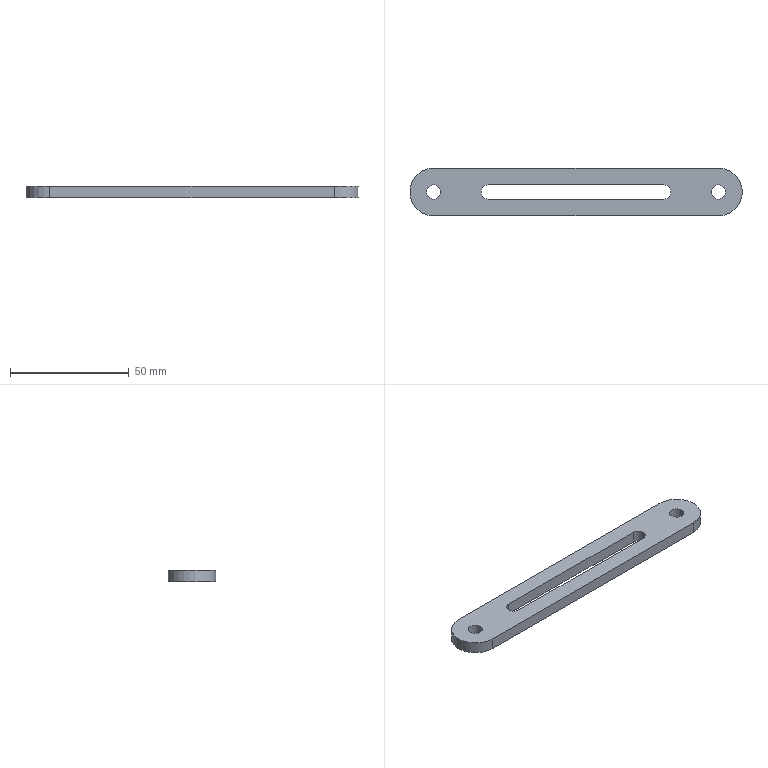Component | NX | LOWER_CONN_PLATE | 1 solid | 12 faces | box 140 x 20 x 5 mm | volume 10927 mm3 | plane 6 | cylinder 6 | commonest cylinder face diameters 6 x4 20 x2
STEP:
#1=CARTESIAN_POINT('',(0.,0.,0.));
#2=DIRECTION('',(0.,0.,1.));
#3=DIRECTION('',(1.,0.,0.));
#4=AXIS2_PLACEMENT_3D('',#1,#2,#3);
#5=CARTESIAN_POINT('',(-37.,3.,2.5));
#6=VERTEX_POINT('',#5);
#7=CARTESIAN_POINT('',(37.,3.,2.5));
#8=VERTEX_POINT('',#7);
#9=CARTESIAN_POINT('',(-40.,3.,2.5));
#10=DIRECTION('',(1.,0.,0.));
#11=VECTOR('',#10,1.);
#12=LINE('',#9,#11);
#13=CARTESIAN_POINT('',(-40.,3.,2.5));
#14=DIRECTION('',(0.,1.,0.));
#15=DIRECTION('',(0.,0.,1.));
#16=AXIS2_PLACEMENT_3D('',#13,#14,#15);
#17=PLANE('',#16);
#18=CARTESIAN_POINT('',(0.,0.));
#19=DIRECTION('',(0.,1.));
#20=VECTOR('',#19,1.);
#21=LINE('',#18,#20);
#22=(GEOMETRIC_REPRESENTATION_CONTEXT(2)PARAMETRIC_REPRESENTATION_CONTEXT()REPRESENTATION_CONTEXT('',''));
#23=DEFINITIONAL_REPRESENTATION('',(#21),#22);
#24=PCURVE('',#17,#23);
#25=CARTESIAN_POINT('',(-60.,0.,2.5));
#26=DIRECTION('',(0.,0.,1.));
#27=DIRECTION('',(1.,0.,0.));
#28=AXIS2_PLACEMENT_3D('',#25,#26,#27);
#29=PLANE('',#28);
#30=CARTESIAN_POINT('',(20.,3.));
#31=DIRECTION('',(1.,0.));
#32=VECTOR('',#31,1.);
#33=LINE('',#30,#32);
#34=(GEOMETRIC_REPRESENTATION_CONTEXT(2)PARAMETRIC_REPRESENTATION_CONTEXT()REPRESENTATION_CONTEXT('',''));
#35=DEFINITIONAL_REPRESENTATION('',(#33),#34);
#36=PCURVE('',#29,#35);
#37=SURFACE_CURVE('',#12,(#24,#36),.PCURVE_S1.);
#38=EDGE_CURVE('',#6,#8,#37,.T.);
#39=ORIENTED_EDGE('',*,*,#38,.F.);
#40=CARTESIAN_POINT('',(-37.,3.,-2.5));
#41=VERTEX_POINT('',#40);
#42=CARTESIAN_POINT('',(-37.,3.,-2.5));
#43=DIRECTION('',(0.,0.,-1.));
#44=VECTOR('',#43,1.);
#45=LINE('',#42,#44);
#46=CARTESIAN_POINT('',(-5.,3.));
#47=DIRECTION('',(-1.,0.));
#48=VECTOR('',#47,1.);
#49=LINE('',#46,#48);
#50=(GEOMETRIC_REPRESENTATION_CONTEXT(2)PARAMETRIC_REPRESENTATION_CONTEXT()REPRESENTATION_CONTEXT('',''));
#51=DEFINITIONAL_REPRESENTATION('',(#49),#50);
#52=PCURVE('',#17,#51);
#53=CARTESIAN_POINT('',(-37.,0.,2.5));
#54=DIRECTION('',(0.,0.,1.));
#55=DIRECTION('',(1.,0.,0.));
#56=AXIS2_PLACEMENT_3D('',#53,#54,#55);
#57=CYLINDRICAL_SURFACE('',#56,3.);
#58=CARTESIAN_POINT('',(1.571,-5.));
#59=DIRECTION('',(0.,-1.));
#60=VECTOR('',#59,1.);
#61=LINE('',#58,#60);
#62=(GEOMETRIC_REPRESENTATION_CONTEXT(2)PARAMETRIC_REPRESENTATION_CONTEXT()REPRESENTATION_CONTEXT('',''));
#63=DEFINITIONAL_REPRESENTATION('',(#61),#62);
#64=PCURVE('',#57,#63);
#65=SURFACE_CURVE('',#45,(#52,#64),.PCURVE_S1.);
#66=EDGE_CURVE('',#6,#41,#65,.T.);
#67=ORIENTED_EDGE('',*,*,#66,.T.);
#68=CARTESIAN_POINT('',(37.,3.,-2.5));
#69=VERTEX_POINT('',#68);
#70=CARTESIAN_POINT('',(-40.,3.,-2.5));
#71=DIRECTION('',(1.,0.,0.));
#72=VECTOR('',#71,1.);
#73=LINE('',#70,#72);
#74=CARTESIAN_POINT('',(-5.,0.));
#75=DIRECTION('',(0.,1.));
#76=VECTOR('',#75,1.);
#77=LINE('',#74,#76);
#78=(GEOMETRIC_REPRESENTATION_CONTEXT(2)PARAMETRIC_REPRESENTATION_CONTEXT()REPRESENTATION_CONTEXT('',''));
#79=DEFINITIONAL_REPRESENTATION('',(#77),#78);
#80=PCURVE('',#17,#79);
#81=CARTESIAN_POINT('',(-60.,0.,-2.5));
#82=DIRECTION('',(0.,0.,1.));
#83=DIRECTION('',(1.,0.,0.));
#84=AXIS2_PLACEMENT_3D('',#81,#82,#83);
#85=PLANE('',#84);
#86=CARTESIAN_POINT('',(20.,3.));
#87=DIRECTION('',(1.,0.));
#88=VECTOR('',#87,1.);
#89=LINE('',#86,#88);
#90=(GEOMETRIC_REPRESENTATION_CONTEXT(2)PARAMETRIC_REPRESENTATION_CONTEXT()REPRESENTATION_CONTEXT('',''));
#91=DEFINITIONAL_REPRESENTATION('',(#89),#90);
#92=PCURVE('',#85,#91);
#93=SURFACE_CURVE('',#73,(#80,#92),.PCURVE_S1.);
#94=EDGE_CURVE('',#41,#69,#93,.T.);
#95=ORIENTED_EDGE('',*,*,#94,.T.);
#96=CARTESIAN_POINT('',(37.,3.,2.5));
#97=DIRECTION('',(0.,0.,1.));
#98=VECTOR('',#97,1.);
#99=LINE('',#96,#98);
#100=CARTESIAN_POINT('',(0.,77.));
#101=DIRECTION('',(1.,0.));
#102=VECTOR('',#101,1.);
#103=LINE('',#100,#102);
#104=(GEOMETRIC_REPRESENTATION_CONTEXT(2)PARAMETRIC_REPRESENTATION_CONTEXT()REPRESENTATION_CONTEXT('',''));
#105=DEFINITIONAL_REPRESENTATION('',(#103),#104);
#106=PCURVE('',#17,#105);
#107=CARTESIAN_POINT('',(37.,0.,2.5));
#108=DIRECTION('',(0.,0.,1.));
#109=DIRECTION('',(1.,0.,0.));
#110=AXIS2_PLACEMENT_3D('',#107,#108,#109);
#111=CYLINDRICAL_SURFACE('',#110,3.);
#112=CARTESIAN_POINT('',(1.571,0.));
#113=DIRECTION('',(0.,1.));
#114=VECTOR('',#113,1.);
#115=LINE('',#112,#114);
#116=(GEOMETRIC_REPRESENTATION_CONTEXT(2)PARAMETRIC_REPRESENTATION_CONTEXT()REPRESENTATION_CONTEXT('',''));
#117=DEFINITIONAL_REPRESENTATION('',(#115),#116);
#118=PCURVE('',#111,#117);
#119=SURFACE_CURVE('',#99,(#106,#118),.PCURVE_S1.);
#120=EDGE_CURVE('',#69,#8,#119,.T.);
#121=ORIENTED_EDGE('',*,*,#120,.T.);
#122=EDGE_LOOP('',(#39,#67,#95,#121));
#123=FACE_BOUND('',#122,.T.);
#124=ADVANCED_FACE('',(#123),#17,.F.);
#125=CARTESIAN_POINT('',(-60.,-10.,-2.5));
#126=VERTEX_POINT('',#125);
#127=CARTESIAN_POINT('',(60.,-10.,-2.5));
#128=VERTEX_POINT('',#127);
#129=CARTESIAN_POINT('',(-70.,-10.,-2.5));
#130=DIRECTION('',(1.,0.,0.));
#131=VECTOR('',#130,1.);
#132=LINE('',#129,#131);
#133=CARTESIAN_POINT('',(-70.,-10.,2.5));
#134=DIRECTION('',(0.,1.,0.));
#135=DIRECTION('',(0.,0.,1.));
#136=AXIS2_PLACEMENT_3D('',#133,#134,#135);
#137=PLANE('',#136);
#138=CARTESIAN_POINT('',(-5.,0.));
#139=DIRECTION('',(0.,1.));
#140=VECTOR('',#139,1.);
#141=LINE('',#138,#140);
#142=(GEOMETRIC_REPRESENTATION_CONTEXT(2)PARAMETRIC_REPRESENTATION_CONTEXT()REPRESENTATION_CONTEXT('',''));
#143=DEFINITIONAL_REPRESENTATION('',(#141),#142);
#144=PCURVE('',#137,#143);
#145=CARTESIAN_POINT('',(-10.,-10.));
#146=DIRECTION('',(1.,0.));
#147=VECTOR('',#146,1.);
#148=LINE('',#145,#147);
#149=(GEOMETRIC_REPRESENTATION_CONTEXT(2)PARAMETRIC_REPRESENTATION_CONTEXT()REPRESENTATION_CONTEXT('',''));
#150=DEFINITIONAL_REPRESENTATION('',(#148),#149);
#151=PCURVE('',#85,#150);
#152=SURFACE_CURVE('',#132,(#144,#151),.PCURVE_S1.);
#153=EDGE_CURVE('',#126,#128,#152,.T.);
#154=ORIENTED_EDGE('',*,*,#153,.T.);
#155=CARTESIAN_POINT('',(60.,-10.,2.5));
#156=VERTEX_POINT('',#155);
#157=CARTESIAN_POINT('',(60.,-10.,2.5));
#158=DIRECTION('',(0.,0.,1.));
#159=VECTOR('',#158,1.);
#160=LINE('',#157,#159);
#161=CARTESIAN_POINT('',(0.,130.));
#162=DIRECTION('',(1.,0.));
#163=VECTOR('',#162,1.);
#164=LINE('',#161,#163);
#165=(GEOMETRIC_REPRESENTATION_CONTEXT(2)PARAMETRIC_REPRESENTATION_CONTEXT()REPRESENTATION_CONTEXT('',''));
#166=DEFINITIONAL_REPRESENTATION('',(#164),#165);
#167=PCURVE('',#137,#166);
#168=CARTESIAN_POINT('',(60.,0.,2.5));
#169=DIRECTION('',(0.,0.,-1.));
#170=DIRECTION('',(-1.,0.,0.));
#171=AXIS2_PLACEMENT_3D('',#168,#169,#170);
#172=CYLINDRICAL_SURFACE('',#171,10.);
#173=CARTESIAN_POINT('',(4.712,0.));
#174=DIRECTION('',(0.,-1.));
#175=VECTOR('',#174,1.);
#176=LINE('',#173,#175);
#177=(GEOMETRIC_REPRESENTATION_CONTEXT(2)PARAMETRIC_REPRESENTATION_CONTEXT()REPRESENTATION_CONTEXT('',''));
#178=DEFINITIONAL_REPRESENTATION('',(#176),#177);
#179=PCURVE('',#172,#178);
#180=SURFACE_CURVE('',#160,(#167,#179),.PCURVE_S1.);
#181=EDGE_CURVE('',#128,#156,#180,.T.);
#182=ORIENTED_EDGE('',*,*,#181,.T.);
#183=CARTESIAN_POINT('',(-60.,-10.,2.5));
#184=VERTEX_POINT('',#183);
#185=CARTESIAN_POINT('',(-70.,-10.,2.5));
#186=DIRECTION('',(1.,0.,0.));
#187=VECTOR('',#186,1.);
#188=LINE('',#185,#187);
#189=CARTESIAN_POINT('',(0.,0.));
#190=DIRECTION('',(0.,1.));
#191=VECTOR('',#190,1.);
#192=LINE('',#189,#191);
#193=(GEOMETRIC_REPRESENTATION_CONTEXT(2)PARAMETRIC_REPRESENTATION_CONTEXT()REPRESENTATION_CONTEXT('',''));
#194=DEFINITIONAL_REPRESENTATION('',(#192),#193);
#195=PCURVE('',#137,#194);
#196=CARTESIAN_POINT('',(-10.,-10.));
#197=DIRECTION('',(1.,0.));
#198=VECTOR('',#197,1.);
#199=LINE('',#196,#198);
#200=(GEOMETRIC_REPRESENTATION_CONTEXT(2)PARAMETRIC_REPRESENTATION_CONTEXT()REPRESENTATION_CONTEXT('',''));
#201=DEFINITIONAL_REPRESENTATION('',(#199),#200);
#202=PCURVE('',#29,#201);
#203=SURFACE_CURVE('',#188,(#195,#202),.PCURVE_S1.);
#204=EDGE_CURVE('',#184,#156,#203,.T.);
#205=ORIENTED_EDGE('',*,*,#204,.F.);
#206=CARTESIAN_POINT('',(-60.,-10.,2.5));
#207=DIRECTION('',(0.,0.,-1.));
#208=VECTOR('',#207,1.);
#209=LINE('',#206,#208);
#210=CARTESIAN_POINT('',(0.,10.));
#211=DIRECTION('',(-1.,0.));
#212=VECTOR('',#211,1.);
#213=LINE('',#210,#212);
#214=(GEOMETRIC_REPRESENTATION_CONTEXT(2)PARAMETRIC_REPRESENTATION_CONTEXT()REPRESENTATION_CONTEXT('',''));
#215=DEFINITIONAL_REPRESENTATION('',(#213),#214);
#216=PCURVE('',#137,#215);
#217=CARTESIAN_POINT('',(-60.,0.,2.5));
#218=DIRECTION('',(0.,0.,-1.));
#219=DIRECTION('',(-1.,0.,0.));
#220=AXIS2_PLACEMENT_3D('',#217,#218,#219);
#221=CYLINDRICAL_SURFACE('',#220,10.);
#222=CARTESIAN_POINT('',(4.712,0.));
#223=DIRECTION('',(0.,1.));
#224=VECTOR('',#223,1.);
#225=LINE('',#222,#224);
#226=(GEOMETRIC_REPRESENTATION_CONTEXT(2)PARAMETRIC_REPRESENTATION_CONTEXT()REPRESENTATION_CONTEXT('',''));
#227=DEFINITIONAL_REPRESENTATION('',(#225),#226);
#228=PCURVE('',#221,#227);
#229=SURFACE_CURVE('',#209,(#216,#228),.PCURVE_S1.);
#230=EDGE_CURVE('',#184,#126,#229,.T.);
#231=ORIENTED_EDGE('',*,*,#230,.T.);
#232=EDGE_LOOP('',(#154,#182,#205,#231));
#233=FACE_BOUND('',#232,.T.);
#234=ADVANCED_FACE('',(#233),#137,.F.);
#235=CARTESIAN_POINT('',(63.,0.,2.5));
#236=VERTEX_POINT('',#235);
#237=CARTESIAN_POINT('',(60.,0.,2.5));
#238=DIRECTION('',(0.,0.,1.));
#239=DIRECTION('',(1.,0.,0.));
#240=AXIS2_PLACEMENT_3D('',#237,#238,#239);
#241=CIRCLE('',#240,3.);
#242=CARTESIAN_POINT('',(60.,0.,2.5));
#243=DIRECTION('',(0.,0.,-1.));
#244=DIRECTION('',(-1.,0.,0.));
#245=AXIS2_PLACEMENT_3D('',#242,#243,#244);
#246=CYLINDRICAL_SURFACE('',#245,3.);
#247=CARTESIAN_POINT('',(9.425,0.));
#248=DIRECTION('',(-1.,0.));
#249=VECTOR('',#248,1.);
#250=LINE('',#247,#249);
#251=(GEOMETRIC_REPRESENTATION_CONTEXT(2)PARAMETRIC_REPRESENTATION_CONTEXT()REPRESENTATION_CONTEXT('',''));
#252=DEFINITIONAL_REPRESENTATION('',(#250),#251);
#253=PCURVE('',#246,#252);
#254=CARTESIAN_POINT('',(120.,0.));
#255=DIRECTION('',(1.,0.));
#256=AXIS2_PLACEMENT_2D('',#254,#255);
#257=CIRCLE('',#256,3.);
#258=(GEOMETRIC_REPRESENTATION_CONTEXT(2)PARAMETRIC_REPRESENTATION_CONTEXT()REPRESENTATION_CONTEXT('',''));
#259=DEFINITIONAL_REPRESENTATION('',(#257),#258);
#260=PCURVE('',#29,#259);
#261=SURFACE_CURVE('',#241,(#253,#260),.PCURVE_S1.);
#262=EDGE_CURVE('',#236,#236,#261,.T.);
#263=ORIENTED_EDGE('',*,*,#262,.F.);
#264=CARTESIAN_POINT('',(63.,0.,-2.5));
#265=VERTEX_POINT('',#264);
#266=CARTESIAN_POINT('',(63.,0.,2.5));
#267=CARTESIAN_POINT('',(63.,0.,-2.5));
#268=B_SPLINE_CURVE_WITH_KNOTS('',1,(#266,#267),.UNSPECIFIED.,.F.,.F.,(2,2),(0.,5.),.PIECEWISE_BEZIER_KNOTS.);
#269=CARTESIAN_POINT('',(9.425,0.));
#270=DIRECTION('',(0.,1.));
#271=VECTOR('',#270,1.);
#272=LINE('',#269,#271);
#273=(GEOMETRIC_REPRESENTATION_CONTEXT(2)PARAMETRIC_REPRESENTATION_CONTEXT()REPRESENTATION_CONTEXT('',''));
#274=DEFINITIONAL_REPRESENTATION('',(#272),#273);
#275=PCURVE('',#246,#274);
#276=CARTESIAN_POINT('',(3.142,0.));
#277=DIRECTION('',(0.,1.));
#278=VECTOR('',#277,1.);
#279=LINE('',#276,#278);
#280=(GEOMETRIC_REPRESENTATION_CONTEXT(2)PARAMETRIC_REPRESENTATION_CONTEXT()REPRESENTATION_CONTEXT('',''));
#281=DEFINITIONAL_REPRESENTATION('',(#279),#280);
#282=PCURVE('',#246,#281);
#283=SEAM_CURVE('',#268,(#275,#282),.PCURVE_S1.);
#284=EDGE_CURVE('',#236,#265,#283,.T.);
#285=ORIENTED_EDGE('',*,*,#284,.T.);
#286=CARTESIAN_POINT('',(60.,0.,-2.5));
#287=DIRECTION('',(0.,0.,1.));
#288=DIRECTION('',(1.,0.,0.));
#289=AXIS2_PLACEMENT_3D('',#286,#287,#288);
#290=CIRCLE('',#289,3.);
#291=CARTESIAN_POINT('',(9.425,5.));
#292=DIRECTION('',(-1.,0.));
#293=VECTOR('',#292,1.);
#294=LINE('',#291,#293);
#295=(GEOMETRIC_REPRESENTATION_CONTEXT(2)PARAMETRIC_REPRESENTATION_CONTEXT()REPRESENTATION_CONTEXT('',''));
#296=DEFINITIONAL_REPRESENTATION('',(#294),#295);
#297=PCURVE('',#246,#296);
#298=CARTESIAN_POINT('',(120.,0.));
#299=DIRECTION('',(1.,0.));
#300=AXIS2_PLACEMENT_2D('',#298,#299);
#301=CIRCLE('',#300,3.);
#302=(GEOMETRIC_REPRESENTATION_CONTEXT(2)PARAMETRIC_REPRESENTATION_CONTEXT()REPRESENTATION_CONTEXT('',''));
#303=DEFINITIONAL_REPRESENTATION('',(#301),#302);
#304=PCURVE('',#85,#303);
#305=SURFACE_CURVE('',#290,(#297,#304),.PCURVE_S1.);
#306=EDGE_CURVE('',#265,#265,#305,.T.);
#307=ORIENTED_EDGE('',*,*,#306,.T.);
#308=ORIENTED_EDGE('',*,*,#284,.F.);
#309=EDGE_LOOP('',(#263,#285,#307,#308));
#310=FACE_BOUND('',#309,.F.);
#311=ADVANCED_FACE('',(#310),#246,.F.);
#312=CARTESIAN_POINT('',(-57.,0.,2.5));
#313=VERTEX_POINT('',#312);
#314=CARTESIAN_POINT('',(-60.,0.,2.5));
#315=DIRECTION('',(0.,0.,1.));
#316=DIRECTION('',(1.,0.,0.));
#317=AXIS2_PLACEMENT_3D('',#314,#315,#316);
#318=CIRCLE('',#317,3.);
#319=CARTESIAN_POINT('',(-60.,0.,2.5));
#320=DIRECTION('',(0.,0.,-1.));
#321=DIRECTION('',(-1.,0.,0.));
#322=AXIS2_PLACEMENT_3D('',#319,#320,#321);
#323=CYLINDRICAL_SURFACE('',#322,3.);
#324=CARTESIAN_POINT('',(9.425,0.));
#325=DIRECTION('',(-1.,0.));
#326=VECTOR('',#325,1.);
#327=LINE('',#324,#326);
#328=(GEOMETRIC_REPRESENTATION_CONTEXT(2)PARAMETRIC_REPRESENTATION_CONTEXT()REPRESENTATION_CONTEXT('',''));
#329=DEFINITIONAL_REPRESENTATION('',(#327),#328);
#330=PCURVE('',#323,#329);
#331=CARTESIAN_POINT('',(0.,0.));
#332=DIRECTION('',(1.,0.));
#333=AXIS2_PLACEMENT_2D('',#331,#332);
#334=CIRCLE('',#333,3.);
#335=(GEOMETRIC_REPRESENTATION_CONTEXT(2)PARAMETRIC_REPRESENTATION_CONTEXT()REPRESENTATION_CONTEXT('',''));
#336=DEFINITIONAL_REPRESENTATION('',(#334),#335);
#337=PCURVE('',#29,#336);
#338=SURFACE_CURVE('',#318,(#330,#337),.PCURVE_S1.);
#339=EDGE_CURVE('',#313,#313,#338,.T.);
#340=ORIENTED_EDGE('',*,*,#339,.F.);
#341=CARTESIAN_POINT('',(-57.,0.,-2.5));
#342=VERTEX_POINT('',#341);
#343=CARTESIAN_POINT('',(-57.,0.,2.5));
#344=CARTESIAN_POINT('',(-57.,0.,-2.5));
#345=B_SPLINE_CURVE_WITH_KNOTS('',1,(#343,#344),.UNSPECIFIED.,.F.,.F.,(2,2),(0.,5.),.PIECEWISE_BEZIER_KNOTS.);
#346=CARTESIAN_POINT('',(9.425,0.));
#347=DIRECTION('',(0.,1.));
#348=VECTOR('',#347,1.);
#349=LINE('',#346,#348);
#350=(GEOMETRIC_REPRESENTATION_CONTEXT(2)PARAMETRIC_REPRESENTATION_CONTEXT()REPRESENTATION_CONTEXT('',''));
#351=DEFINITIONAL_REPRESENTATION('',(#349),#350);
#352=PCURVE('',#323,#351);
#353=CARTESIAN_POINT('',(3.142,0.));
#354=DIRECTION('',(0.,1.));
#355=VECTOR('',#354,1.);
#356=LINE('',#353,#355);
#357=(GEOMETRIC_REPRESENTATION_CONTEXT(2)PARAMETRIC_REPRESENTATION_CONTEXT()REPRESENTATION_CONTEXT('',''));
#358=DEFINITIONAL_REPRESENTATION('',(#356),#357);
#359=PCURVE('',#323,#358);
#360=SEAM_CURVE('',#345,(#352,#359),.PCURVE_S1.);
#361=EDGE_CURVE('',#313,#342,#360,.T.);
#362=ORIENTED_EDGE('',*,*,#361,.T.);
#363=CARTESIAN_POINT('',(-60.,0.,-2.5));
#364=DIRECTION('',(0.,0.,1.));
#365=DIRECTION('',(1.,0.,0.));
#366=AXIS2_PLACEMENT_3D('',#363,#364,#365);
#367=CIRCLE('',#366,3.);
#368=CARTESIAN_POINT('',(9.425,5.));
#369=DIRECTION('',(-1.,0.));
#370=VECTOR('',#369,1.);
#371=LINE('',#368,#370);
#372=(GEOMETRIC_REPRESENTATION_CONTEXT(2)PARAMETRIC_REPRESENTATION_CONTEXT()REPRESENTATION_CONTEXT('',''));
#373=DEFINITIONAL_REPRESENTATION('',(#371),#372);
#374=PCURVE('',#323,#373);
#375=CARTESIAN_POINT('',(0.,0.));
#376=DIRECTION('',(1.,0.));
#377=AXIS2_PLACEMENT_2D('',#375,#376);
#378=CIRCLE('',#377,3.);
#379=(GEOMETRIC_REPRESENTATION_CONTEXT(2)PARAMETRIC_REPRESENTATION_CONTEXT()REPRESENTATION_CONTEXT('',''));
#380=DEFINITIONAL_REPRESENTATION('',(#378),#379);
#381=PCURVE('',#85,#380);
#382=SURFACE_CURVE('',#367,(#374,#381),.PCURVE_S1.);
#383=EDGE_CURVE('',#342,#342,#382,.T.);
#384=ORIENTED_EDGE('',*,*,#383,.T.);
#385=ORIENTED_EDGE('',*,*,#361,.F.);
#386=EDGE_LOOP('',(#340,#362,#384,#385));
#387=FACE_BOUND('',#386,.F.);
#388=ADVANCED_FACE('',(#387),#323,.F.);
#389=CARTESIAN_POINT('',(60.,10.,2.5));
#390=VERTEX_POINT('',#389);
#391=CARTESIAN_POINT('',(-60.,10.,2.5));
#392=VERTEX_POINT('',#391);
#393=CARTESIAN_POINT('',(70.,10.,2.5));
#394=DIRECTION('',(-1.,0.,0.));
#395=VECTOR('',#394,1.);
#396=LINE('',#393,#395);
#397=CARTESIAN_POINT('',(70.,10.,2.5));
#398=DIRECTION('',(0.,-1.,0.));
#399=DIRECTION('',(0.,0.,-1.));
#400=AXIS2_PLACEMENT_3D('',#397,#398,#399);
#401=PLANE('',#400);
#402=CARTESIAN_POINT('',(0.,0.));
#403=DIRECTION('',(0.,-1.));
#404=VECTOR('',#403,1.);
#405=LINE('',#402,#404);
#406=(GEOMETRIC_REPRESENTATION_CONTEXT(2)PARAMETRIC_REPRESENTATION_CONTEXT()REPRESENTATION_CONTEXT('',''));
#407=DEFINITIONAL_REPRESENTATION('',(#405),#406);
#408=PCURVE('',#401,#407);
#409=CARTESIAN_POINT('',(130.,10.));
#410=DIRECTION('',(-1.,0.));
#411=VECTOR('',#410,1.);
#412=LINE('',#409,#411);
#413=(GEOMETRIC_REPRESENTATION_CONTEXT(2)PARAMETRIC_REPRESENTATION_CONTEXT()REPRESENTATION_CONTEXT('',''));
#414=DEFINITIONAL_REPRESENTATION('',(#412),#413);
#415=PCURVE('',#29,#414);
#416=SURFACE_CURVE('',#396,(#408,#415),.PCURVE_S1.);
#417=EDGE_CURVE('',#390,#392,#416,.T.);
#418=ORIENTED_EDGE('',*,*,#417,.F.);
#419=CARTESIAN_POINT('',(60.,10.,-2.5));
#420=VERTEX_POINT('',#419);
#421=CARTESIAN_POINT('',(60.,10.,2.5));
#422=DIRECTION('',(0.,0.,-1.));
#423=VECTOR('',#422,1.);
#424=LINE('',#421,#423);
#425=CARTESIAN_POINT('',(0.,-10.));
#426=DIRECTION('',(1.,0.));
#427=VECTOR('',#426,1.);
#428=LINE('',#425,#427);
#429=(GEOMETRIC_REPRESENTATION_CONTEXT(2)PARAMETRIC_REPRESENTATION_CONTEXT()REPRESENTATION_CONTEXT('',''));
#430=DEFINITIONAL_REPRESENTATION('',(#428),#429);
#431=PCURVE('',#401,#430);
#432=CARTESIAN_POINT('',(1.571,0.));
#433=DIRECTION('',(0.,1.));
#434=VECTOR('',#433,1.);
#435=LINE('',#432,#434);
#436=(GEOMETRIC_REPRESENTATION_CONTEXT(2)PARAMETRIC_REPRESENTATION_CONTEXT()REPRESENTATION_CONTEXT('',''));
#437=DEFINITIONAL_REPRESENTATION('',(#435),#436);
#438=PCURVE('',#172,#437);
#439=SURFACE_CURVE('',#424,(#431,#438),.PCURVE_S1.);
#440=EDGE_CURVE('',#390,#420,#439,.T.);
#441=ORIENTED_EDGE('',*,*,#440,.T.);
#442=CARTESIAN_POINT('',(-60.,10.,-2.5));
#443=VERTEX_POINT('',#442);
#444=CARTESIAN_POINT('',(70.,10.,-2.5));
#445=DIRECTION('',(-1.,0.,0.));
#446=VECTOR('',#445,1.);
#447=LINE('',#444,#446);
#448=CARTESIAN_POINT('',(5.,0.));
#449=DIRECTION('',(0.,-1.));
#450=VECTOR('',#449,1.);
#451=LINE('',#448,#450);
#452=(GEOMETRIC_REPRESENTATION_CONTEXT(2)PARAMETRIC_REPRESENTATION_CONTEXT()REPRESENTATION_CONTEXT('',''));
#453=DEFINITIONAL_REPRESENTATION('',(#451),#452);
#454=PCURVE('',#401,#453);
#455=CARTESIAN_POINT('',(130.,10.));
#456=DIRECTION('',(-1.,0.));
#457=VECTOR('',#456,1.);
#458=LINE('',#455,#457);
#459=(GEOMETRIC_REPRESENTATION_CONTEXT(2)PARAMETRIC_REPRESENTATION_CONTEXT()REPRESENTATION_CONTEXT('',''));
#460=DEFINITIONAL_REPRESENTATION('',(#458),#459);
#461=PCURVE('',#85,#460);
#462=SURFACE_CURVE('',#447,(#454,#461),.PCURVE_S1.);
#463=EDGE_CURVE('',#420,#443,#462,.T.);
#464=ORIENTED_EDGE('',*,*,#463,.T.);
#465=CARTESIAN_POINT('',(-60.,10.,2.5));
#466=DIRECTION('',(0.,0.,1.));
#467=VECTOR('',#466,1.);
#468=LINE('',#465,#467);
#469=CARTESIAN_POINT('',(0.,-130.));
#470=DIRECTION('',(-1.,0.));
#471=VECTOR('',#470,1.);
#472=LINE('',#469,#471);
#473=(GEOMETRIC_REPRESENTATION_CONTEXT(2)PARAMETRIC_REPRESENTATION_CONTEXT()REPRESENTATION_CONTEXT('',''));
#474=DEFINITIONAL_REPRESENTATION('',(#472),#473);
#475=PCURVE('',#401,#474);
#476=CARTESIAN_POINT('',(7.854,0.));
#477=DIRECTION('',(0.,-1.));
#478=VECTOR('',#477,1.);
#479=LINE('',#476,#478);
#480=(GEOMETRIC_REPRESENTATION_CONTEXT(2)PARAMETRIC_REPRESENTATION_CONTEXT()REPRESENTATION_CONTEXT('',''));
#481=DEFINITIONAL_REPRESENTATION('',(#479),#480);
#482=PCURVE('',#221,#481);
#483=SURFACE_CURVE('',#468,(#475,#482),.PCURVE_S1.);
#484=EDGE_CURVE('',#443,#392,#483,.T.);
#485=ORIENTED_EDGE('',*,*,#484,.T.);
#486=EDGE_LOOP('',(#418,#441,#464,#485));
#487=FACE_BOUND('',#486,.T.);
#488=ADVANCED_FACE('',(#487),#401,.F.);
#489=CARTESIAN_POINT('',(37.,-3.,-2.5));
#490=VERTEX_POINT('',#489);
#491=CARTESIAN_POINT('',(-37.,-3.,-2.5));
#492=VERTEX_POINT('',#491);
#493=CARTESIAN_POINT('',(40.,-3.,-2.5));
#494=DIRECTION('',(-1.,0.,0.));
#495=VECTOR('',#494,1.);
#496=LINE('',#493,#495);
#497=CARTESIAN_POINT('',(40.,-3.,2.5));
#498=DIRECTION('',(0.,-1.,0.));
#499=DIRECTION('',(0.,0.,-1.));
#500=AXIS2_PLACEMENT_3D('',#497,#498,#499);
#501=PLANE('',#500);
#502=CARTESIAN_POINT('',(5.,0.));
#503=DIRECTION('',(0.,-1.));
#504=VECTOR('',#503,1.);
#505=LINE('',#502,#504);
#506=(GEOMETRIC_REPRESENTATION_CONTEXT(2)PARAMETRIC_REPRESENTATION_CONTEXT()REPRESENTATION_CONTEXT('',''));
#507=DEFINITIONAL_REPRESENTATION('',(#505),#506);
#508=PCURVE('',#501,#507);
#509=CARTESIAN_POINT('',(100.,-3.));
#510=DIRECTION('',(-1.,0.));
#511=VECTOR('',#510,1.);
#512=LINE('',#509,#511);
#513=(GEOMETRIC_REPRESENTATION_CONTEXT(2)PARAMETRIC_REPRESENTATION_CONTEXT()REPRESENTATION_CONTEXT('',''));
#514=DEFINITIONAL_REPRESENTATION('',(#512),#513);
#515=PCURVE('',#85,#514);
#516=SURFACE_CURVE('',#496,(#508,#515),.PCURVE_S1.);
#517=EDGE_CURVE('',#490,#492,#516,.T.);
#518=ORIENTED_EDGE('',*,*,#517,.T.);
#519=CARTESIAN_POINT('',(-37.,-3.,2.5));
#520=VERTEX_POINT('',#519);
#521=CARTESIAN_POINT('',(-37.,-3.,2.5));
#522=DIRECTION('',(0.,0.,1.));
#523=VECTOR('',#522,1.);
#524=LINE('',#521,#523);
#525=CARTESIAN_POINT('',(0.,-77.));
#526=DIRECTION('',(-1.,0.));
#527=VECTOR('',#526,1.);
#528=LINE('',#525,#527);
#529=(GEOMETRIC_REPRESENTATION_CONTEXT(2)PARAMETRIC_REPRESENTATION_CONTEXT()REPRESENTATION_CONTEXT('',''));
#530=DEFINITIONAL_REPRESENTATION('',(#528),#529);
#531=PCURVE('',#501,#530);
#532=CARTESIAN_POINT('',(4.712,0.));
#533=DIRECTION('',(0.,1.));
#534=VECTOR('',#533,1.);
#535=LINE('',#532,#534);
#536=(GEOMETRIC_REPRESENTATION_CONTEXT(2)PARAMETRIC_REPRESENTATION_CONTEXT()REPRESENTATION_CONTEXT('',''));
#537=DEFINITIONAL_REPRESENTATION('',(#535),#536);
#538=PCURVE('',#57,#537);
#539=SURFACE_CURVE('',#524,(#531,#538),.PCURVE_S1.);
#540=EDGE_CURVE('',#492,#520,#539,.T.);
#541=ORIENTED_EDGE('',*,*,#540,.T.);
#542=CARTESIAN_POINT('',(37.,-3.,2.5));
#543=VERTEX_POINT('',#542);
#544=CARTESIAN_POINT('',(40.,-3.,2.5));
#545=DIRECTION('',(-1.,0.,0.));
#546=VECTOR('',#545,1.);
#547=LINE('',#544,#546);
#548=CARTESIAN_POINT('',(0.,0.));
#549=DIRECTION('',(0.,-1.));
#550=VECTOR('',#549,1.);
#551=LINE('',#548,#550);
#552=(GEOMETRIC_REPRESENTATION_CONTEXT(2)PARAMETRIC_REPRESENTATION_CONTEXT()REPRESENTATION_CONTEXT('',''));
#553=DEFINITIONAL_REPRESENTATION('',(#551),#552);
#554=PCURVE('',#501,#553);
#555=CARTESIAN_POINT('',(100.,-3.));
#556=DIRECTION('',(-1.,0.));
#557=VECTOR('',#556,1.);
#558=LINE('',#555,#557);
#559=(GEOMETRIC_REPRESENTATION_CONTEXT(2)PARAMETRIC_REPRESENTATION_CONTEXT()REPRESENTATION_CONTEXT('',''));
#560=DEFINITIONAL_REPRESENTATION('',(#558),#559);
#561=PCURVE('',#29,#560);
#562=SURFACE_CURVE('',#547,(#554,#561),.PCURVE_S1.);
#563=EDGE_CURVE('',#543,#520,#562,.T.);
#564=ORIENTED_EDGE('',*,*,#563,.F.);
#565=CARTESIAN_POINT('',(37.,-3.,-2.5));
#566=DIRECTION('',(0.,0.,-1.));
#567=VECTOR('',#566,1.);
#568=LINE('',#565,#567);
#569=CARTESIAN_POINT('',(5.,-3.));
#570=DIRECTION('',(1.,0.));
#571=VECTOR('',#570,1.);
#572=LINE('',#569,#571);
#573=(GEOMETRIC_REPRESENTATION_CONTEXT(2)PARAMETRIC_REPRESENTATION_CONTEXT()REPRESENTATION_CONTEXT('',''));
#574=DEFINITIONAL_REPRESENTATION('',(#572),#573);
#575=PCURVE('',#501,#574);
#576=CARTESIAN_POINT('',(-1.571,-5.));
#577=DIRECTION('',(0.,-1.));
#578=VECTOR('',#577,1.);
#579=LINE('',#576,#578);
#580=(GEOMETRIC_REPRESENTATION_CONTEXT(2)PARAMETRIC_REPRESENTATION_CONTEXT()REPRESENTATION_CONTEXT('',''));
#581=DEFINITIONAL_REPRESENTATION('',(#579),#580);
#582=PCURVE('',#111,#581);
#583=SURFACE_CURVE('',#568,(#575,#582),.PCURVE_S1.);
#584=EDGE_CURVE('',#543,#490,#583,.T.);
#585=ORIENTED_EDGE('',*,*,#584,.T.);
#586=EDGE_LOOP('',(#518,#541,#564,#585));
#587=FACE_BOUND('',#586,.T.);
#588=ADVANCED_FACE('',(#587),#501,.F.);
#589=CARTESIAN_POINT('',(60.,0.,2.5));
#590=DIRECTION('',(0.,0.,1.));
#591=DIRECTION('',(1.,0.,0.));
#592=AXIS2_PLACEMENT_3D('',#589,#590,#591);
#593=CIRCLE('',#592,10.);
#594=CARTESIAN_POINT('',(120.,0.));
#595=DIRECTION('',(1.,0.));
#596=AXIS2_PLACEMENT_2D('',#594,#595);
#597=CIRCLE('',#596,10.);
#598=(GEOMETRIC_REPRESENTATION_CONTEXT(2)PARAMETRIC_REPRESENTATION_CONTEXT()REPRESENTATION_CONTEXT('',''));
#599=DEFINITIONAL_REPRESENTATION('',(#597),#598);
#600=PCURVE('',#29,#599);
#601=CARTESIAN_POINT('',(9.425,0.));
#602=DIRECTION('',(-1.,0.));
#603=VECTOR('',#602,1.);
#604=LINE('',#601,#603);
#605=(GEOMETRIC_REPRESENTATION_CONTEXT(2)PARAMETRIC_REPRESENTATION_CONTEXT()REPRESENTATION_CONTEXT('',''));
#606=DEFINITIONAL_REPRESENTATION('',(#604),#605);
#607=PCURVE('',#172,#606);
#608=SURFACE_CURVE('',#593,(#600,#607),.PCURVE_S1.);
#609=EDGE_CURVE('',#156,#390,#608,.T.);
#610=ORIENTED_EDGE('',*,*,#609,.T.);
#611=ORIENTED_EDGE('',*,*,#417,.T.);
#612=CARTESIAN_POINT('',(-60.,0.,2.5));
#613=DIRECTION('',(0.,0.,1.));
#614=DIRECTION('',(1.,0.,0.));
#615=AXIS2_PLACEMENT_3D('',#612,#613,#614);
#616=CIRCLE('',#615,10.);
#617=CARTESIAN_POINT('',(0.,0.));
#618=DIRECTION('',(1.,0.));
#619=AXIS2_PLACEMENT_2D('',#617,#618);
#620=CIRCLE('',#619,10.);
#621=(GEOMETRIC_REPRESENTATION_CONTEXT(2)PARAMETRIC_REPRESENTATION_CONTEXT()REPRESENTATION_CONTEXT('',''));
#622=DEFINITIONAL_REPRESENTATION('',(#620),#621);
#623=PCURVE('',#29,#622);
#624=CARTESIAN_POINT('',(9.425,0.));
#625=DIRECTION('',(-1.,0.));
#626=VECTOR('',#625,1.);
#627=LINE('',#624,#626);
#628=(GEOMETRIC_REPRESENTATION_CONTEXT(2)PARAMETRIC_REPRESENTATION_CONTEXT()REPRESENTATION_CONTEXT('',''));
#629=DEFINITIONAL_REPRESENTATION('',(#627),#628);
#630=PCURVE('',#221,#629);
#631=SURFACE_CURVE('',#616,(#623,#630),.PCURVE_S1.);
#632=EDGE_CURVE('',#392,#184,#631,.T.);
#633=ORIENTED_EDGE('',*,*,#632,.T.);
#634=ORIENTED_EDGE('',*,*,#204,.T.);
#635=EDGE_LOOP('',(#610,#611,#633,#634));
#636=FACE_BOUND('',#635,.T.);
#637=ORIENTED_EDGE('',*,*,#339,.F.);
#638=EDGE_LOOP('',(#637));
#639=FACE_BOUND('',#638,.T.);
#640=ORIENTED_EDGE('',*,*,#262,.F.);
#641=EDGE_LOOP('',(#640));
#642=FACE_BOUND('',#641,.T.);
#643=ORIENTED_EDGE('',*,*,#563,.T.);
#644=CARTESIAN_POINT('',(-37.,0.,2.5));
#645=DIRECTION('',(0.,0.,-1.));
#646=DIRECTION('',(1.,0.,0.));
#647=AXIS2_PLACEMENT_3D('',#644,#645,#646);
#648=CIRCLE('',#647,3.);
#649=CARTESIAN_POINT('',(26.,0.));
#650=CARTESIAN_POINT('',(26.,-5.196));
#651=CARTESIAN_POINT('',(21.5,-2.598));
#652=CARTESIAN_POINT('',(17.,0.));
#653=CARTESIAN_POINT('',(21.5,2.598));
#654=CARTESIAN_POINT('',(26.,5.196));
#655=CARTESIAN_POINT('',(26.,0.));
#656=(BOUNDED_CURVE()B_SPLINE_CURVE(2,(#649,#650,#651,#652,#653,#654,#655),.UNSPECIFIED.,.T.,.F.)B_SPLINE_CURVE_WITH_KNOTS((1,2,2,2,2,1),(-2.094,0.,2.094,4.189,6.283,8.378),.UNSPECIFIED.)CURVE()GEOMETRIC_REPRESENTATION_ITEM()RATIONAL_B_SPLINE_CURVE((1.,0.5,1.,0.5,1.,0.5,1.))REPRESENTATION_ITEM(''));
#657=(GEOMETRIC_REPRESENTATION_CONTEXT(2)PARAMETRIC_REPRESENTATION_CONTEXT()REPRESENTATION_CONTEXT('',''));
#658=DEFINITIONAL_REPRESENTATION('',(#656),#657);
#659=PCURVE('',#29,#658);
#660=CARTESIAN_POINT('',(6.283,0.));
#661=DIRECTION('',(-1.,0.));
#662=VECTOR('',#661,1.);
#663=LINE('',#660,#662);
#664=(GEOMETRIC_REPRESENTATION_CONTEXT(2)PARAMETRIC_REPRESENTATION_CONTEXT()REPRESENTATION_CONTEXT('',''));
#665=DEFINITIONAL_REPRESENTATION('',(#663),#664);
#666=PCURVE('',#57,#665);
#667=SURFACE_CURVE('',#648,(#659,#666),.PCURVE_S1.);
#668=EDGE_CURVE('',#520,#6,#667,.T.);
#669=ORIENTED_EDGE('',*,*,#668,.T.);
#670=ORIENTED_EDGE('',*,*,#38,.T.);
#671=CARTESIAN_POINT('',(37.,0.,2.5));
#672=DIRECTION('',(0.,0.,-1.));
#673=DIRECTION('',(1.,0.,0.));
#674=AXIS2_PLACEMENT_3D('',#671,#672,#673);
#675=CIRCLE('',#674,3.);
#676=CARTESIAN_POINT('',(100.,0.));
#677=CARTESIAN_POINT('',(100.,-5.196));
#678=CARTESIAN_POINT('',(95.5,-2.598));
#679=CARTESIAN_POINT('',(91.,-0.));
#680=CARTESIAN_POINT('',(95.5,2.598));
#681=CARTESIAN_POINT('',(100.,5.196));
#682=CARTESIAN_POINT('',(100.,0.));
#683=(BOUNDED_CURVE()B_SPLINE_CURVE(2,(#676,#677,#678,#679,#680,#681,#682),.UNSPECIFIED.,.T.,.F.)B_SPLINE_CURVE_WITH_KNOTS((1,2,2,2,2,1),(-2.094,0.,2.094,4.189,6.283,8.378),.UNSPECIFIED.)CURVE()GEOMETRIC_REPRESENTATION_ITEM()RATIONAL_B_SPLINE_CURVE((1.,0.5,1.,0.5,1.,0.5,1.))REPRESENTATION_ITEM(''));
#684=(GEOMETRIC_REPRESENTATION_CONTEXT(2)PARAMETRIC_REPRESENTATION_CONTEXT()REPRESENTATION_CONTEXT('',''));
#685=DEFINITIONAL_REPRESENTATION('',(#683),#684);
#686=PCURVE('',#29,#685);
#687=CARTESIAN_POINT('',(6.283,0.));
#688=DIRECTION('',(-1.,0.));
#689=VECTOR('',#688,1.);
#690=LINE('',#687,#689);
#691=(GEOMETRIC_REPRESENTATION_CONTEXT(2)PARAMETRIC_REPRESENTATION_CONTEXT()REPRESENTATION_CONTEXT('',''));
#692=DEFINITIONAL_REPRESENTATION('',(#690),#691);
#693=PCURVE('',#111,#692);
#694=SURFACE_CURVE('',#675,(#686,#693),.PCURVE_S1.);
#695=EDGE_CURVE('',#8,#543,#694,.T.);
#696=ORIENTED_EDGE('',*,*,#695,.T.);
#697=EDGE_LOOP('',(#643,#669,#670,#696));
#698=FACE_BOUND('',#697,.T.);
#699=ADVANCED_FACE('',(#636,#639,#642,#698),#29,.T.);
#700=ORIENTED_EDGE('',*,*,#463,.F.);
#701=CARTESIAN_POINT('',(60.,0.,-2.5));
#702=DIRECTION('',(0.,0.,-1.));
#703=DIRECTION('',(1.,0.,0.));
#704=AXIS2_PLACEMENT_3D('',#701,#702,#703);
#705=CIRCLE('',#704,10.);
#706=CARTESIAN_POINT('',(130.,0.));
#707=CARTESIAN_POINT('',(130.,-17.321));
#708=CARTESIAN_POINT('',(115.,-8.66));
#709=CARTESIAN_POINT('',(100.,-0.));
#710=CARTESIAN_POINT('',(115.,8.66));
#711=CARTESIAN_POINT('',(130.,17.321));
#712=CARTESIAN_POINT('',(130.,0.));
#713=(BOUNDED_CURVE()B_SPLINE_CURVE(2,(#706,#707,#708,#709,#710,#711,#712),.UNSPECIFIED.,.T.,.F.)B_SPLINE_CURVE_WITH_KNOTS((1,2,2,2,2,1),(-2.094,0.,2.094,4.189,6.283,8.378),.UNSPECIFIED.)CURVE()GEOMETRIC_REPRESENTATION_ITEM()RATIONAL_B_SPLINE_CURVE((1.,0.5,1.,0.5,1.,0.5,1.))REPRESENTATION_ITEM(''));
#714=(GEOMETRIC_REPRESENTATION_CONTEXT(2)PARAMETRIC_REPRESENTATION_CONTEXT()REPRESENTATION_CONTEXT('',''));
#715=DEFINITIONAL_REPRESENTATION('',(#713),#714);
#716=PCURVE('',#85,#715);
#717=CARTESIAN_POINT('',(-3.142,5.));
#718=DIRECTION('',(1.,0.));
#719=VECTOR('',#718,1.);
#720=LINE('',#717,#719);
#721=(GEOMETRIC_REPRESENTATION_CONTEXT(2)PARAMETRIC_REPRESENTATION_CONTEXT()REPRESENTATION_CONTEXT('',''));
#722=DEFINITIONAL_REPRESENTATION('',(#720),#721);
#723=PCURVE('',#172,#722);
#724=SURFACE_CURVE('',#705,(#716,#723),.PCURVE_S1.);
#725=EDGE_CURVE('',#420,#128,#724,.T.);
#726=ORIENTED_EDGE('',*,*,#725,.T.);
#727=ORIENTED_EDGE('',*,*,#153,.F.);
#728=CARTESIAN_POINT('',(-60.,0.,-2.5));
#729=DIRECTION('',(0.,0.,-1.));
#730=DIRECTION('',(1.,0.,0.));
#731=AXIS2_PLACEMENT_3D('',#728,#729,#730);
#732=CIRCLE('',#731,10.);
#733=CARTESIAN_POINT('',(10.,0.));
#734=CARTESIAN_POINT('',(10.,-17.321));
#735=CARTESIAN_POINT('',(-5.,-8.66));
#736=CARTESIAN_POINT('',(-20.,-0.));
#737=CARTESIAN_POINT('',(-5.,8.66));
#738=CARTESIAN_POINT('',(10.,17.321));
#739=CARTESIAN_POINT('',(10.,0.));
#740=(BOUNDED_CURVE()B_SPLINE_CURVE(2,(#733,#734,#735,#736,#737,#738,#739),.UNSPECIFIED.,.T.,.F.)B_SPLINE_CURVE_WITH_KNOTS((1,2,2,2,2,1),(-2.094,0.,2.094,4.189,6.283,8.378),.UNSPECIFIED.)CURVE()GEOMETRIC_REPRESENTATION_ITEM()RATIONAL_B_SPLINE_CURVE((1.,0.5,1.,0.5,1.,0.5,1.))REPRESENTATION_ITEM(''));
#741=(GEOMETRIC_REPRESENTATION_CONTEXT(2)PARAMETRIC_REPRESENTATION_CONTEXT()REPRESENTATION_CONTEXT('',''));
#742=DEFINITIONAL_REPRESENTATION('',(#740),#741);
#743=PCURVE('',#85,#742);
#744=CARTESIAN_POINT('',(3.142,5.));
#745=DIRECTION('',(1.,0.));
#746=VECTOR('',#745,1.);
#747=LINE('',#744,#746);
#748=(GEOMETRIC_REPRESENTATION_CONTEXT(2)PARAMETRIC_REPRESENTATION_CONTEXT()REPRESENTATION_CONTEXT('',''));
#749=DEFINITIONAL_REPRESENTATION('',(#747),#748);
#750=PCURVE('',#221,#749);
#751=SURFACE_CURVE('',#732,(#743,#750),.PCURVE_S1.);
#752=EDGE_CURVE('',#126,#443,#751,.T.);
#753=ORIENTED_EDGE('',*,*,#752,.T.);
#754=EDGE_LOOP('',(#700,#726,#727,#753));
#755=FACE_BOUND('',#754,.T.);
#756=ORIENTED_EDGE('',*,*,#383,.T.);
#757=EDGE_LOOP('',(#756));
#758=FACE_BOUND('',#757,.T.);
#759=ORIENTED_EDGE('',*,*,#306,.T.);
#760=EDGE_LOOP('',(#759));
#761=FACE_BOUND('',#760,.T.);
#762=CARTESIAN_POINT('',(-37.,0.,-2.5));
#763=DIRECTION('',(0.,0.,1.));
#764=DIRECTION('',(1.,0.,0.));
#765=AXIS2_PLACEMENT_3D('',#762,#763,#764);
#766=CIRCLE('',#765,3.);
#767=CARTESIAN_POINT('',(23.,0.));
#768=DIRECTION('',(1.,0.));
#769=AXIS2_PLACEMENT_2D('',#767,#768);
#770=CIRCLE('',#769,3.);
#771=(GEOMETRIC_REPRESENTATION_CONTEXT(2)PARAMETRIC_REPRESENTATION_CONTEXT()REPRESENTATION_CONTEXT('',''));
#772=DEFINITIONAL_REPRESENTATION('',(#770),#771);
#773=PCURVE('',#85,#772);
#774=CARTESIAN_POINT('',(0.,-5.));
#775=DIRECTION('',(1.,0.));
#776=VECTOR('',#775,1.);
#777=LINE('',#774,#776);
#778=(GEOMETRIC_REPRESENTATION_CONTEXT(2)PARAMETRIC_REPRESENTATION_CONTEXT()REPRESENTATION_CONTEXT('',''));
#779=DEFINITIONAL_REPRESENTATION('',(#777),#778);
#780=PCURVE('',#57,#779);
#781=SURFACE_CURVE('',#766,(#773,#780),.PCURVE_S1.);
#782=EDGE_CURVE('',#41,#492,#781,.T.);
#783=ORIENTED_EDGE('',*,*,#782,.T.);
#784=ORIENTED_EDGE('',*,*,#517,.F.);
#785=CARTESIAN_POINT('',(37.,0.,-2.5));
#786=DIRECTION('',(0.,0.,1.));
#787=DIRECTION('',(1.,0.,0.));
#788=AXIS2_PLACEMENT_3D('',#785,#786,#787);
#789=CIRCLE('',#788,3.);
#790=CARTESIAN_POINT('',(97.,0.));
#791=DIRECTION('',(1.,0.));
#792=AXIS2_PLACEMENT_2D('',#790,#791);
#793=CIRCLE('',#792,3.);
#794=(GEOMETRIC_REPRESENTATION_CONTEXT(2)PARAMETRIC_REPRESENTATION_CONTEXT()REPRESENTATION_CONTEXT('',''));
#795=DEFINITIONAL_REPRESENTATION('',(#793),#794);
#796=PCURVE('',#85,#795);
#797=CARTESIAN_POINT('',(-6.283,-5.));
#798=DIRECTION('',(1.,0.));
#799=VECTOR('',#798,1.);
#800=LINE('',#797,#799);
#801=(GEOMETRIC_REPRESENTATION_CONTEXT(2)PARAMETRIC_REPRESENTATION_CONTEXT()REPRESENTATION_CONTEXT('',''));
#802=DEFINITIONAL_REPRESENTATION('',(#800),#801);
#803=PCURVE('',#111,#802);
#804=SURFACE_CURVE('',#789,(#796,#803),.PCURVE_S1.);
#805=EDGE_CURVE('',#490,#69,#804,.T.);
#806=ORIENTED_EDGE('',*,*,#805,.T.);
#807=ORIENTED_EDGE('',*,*,#94,.F.);
#808=EDGE_LOOP('',(#783,#784,#806,#807));
#809=FACE_BOUND('',#808,.T.);
#810=ADVANCED_FACE('',(#755,#758,#761,#809),#85,.F.);
#811=ORIENTED_EDGE('',*,*,#668,.T.);
#812=ORIENTED_EDGE('',*,*,#66,.T.);
#813=ORIENTED_EDGE('',*,*,#782,.T.);
#814=ORIENTED_EDGE('',*,*,#540,.T.);
#815=EDGE_LOOP('',(#811,#812,#813,#814));
#816=FACE_BOUND('',#815,.F.);
#817=ADVANCED_FACE('',(#816),#57,.F.);
#818=ORIENTED_EDGE('',*,*,#695,.T.);
#819=ORIENTED_EDGE('',*,*,#584,.T.);
#820=ORIENTED_EDGE('',*,*,#805,.T.);
#821=ORIENTED_EDGE('',*,*,#120,.T.);
#822=EDGE_LOOP('',(#818,#819,#820,#821));
#823=FACE_BOUND('',#822,.F.);
#824=ADVANCED_FACE('',(#823),#111,.F.);
#825=ORIENTED_EDGE('',*,*,#725,.F.);
#826=ORIENTED_EDGE('',*,*,#440,.F.);
#827=ORIENTED_EDGE('',*,*,#609,.F.);
#828=ORIENTED_EDGE('',*,*,#181,.F.);
#829=EDGE_LOOP('',(#825,#826,#827,#828));
#830=FACE_BOUND('',#829,.T.);
#831=ADVANCED_FACE('',(#830),#172,.T.);
#832=ORIENTED_EDGE('',*,*,#230,.F.);
#833=ORIENTED_EDGE('',*,*,#632,.F.);
#834=ORIENTED_EDGE('',*,*,#484,.F.);
#835=ORIENTED_EDGE('',*,*,#752,.F.);
#836=EDGE_LOOP('',(#832,#833,#834,#835));
#837=FACE_BOUND('',#836,.T.);
#838=ADVANCED_FACE('',(#837),#221,.T.);
#839=CLOSED_SHELL('',(#124,#234,#311,#388,#488,#588,#699,#810,#817,#824,#831,#838));
#840=MANIFOLD_SOLID_BREP('',#839);
#841=(LENGTH_UNIT()NAMED_UNIT(*)SI_UNIT(.MILLI.,.METRE.));
#842=UNCERTAINTY_MEASURE_WITH_UNIT(LENGTH_MEASURE(0.000002),#841,'','');
#843=(NAMED_UNIT(*)PLANE_ANGLE_UNIT()SI_UNIT($,.RADIAN.));
#844=(NAMED_UNIT(*)SI_UNIT($,.STERADIAN.)SOLID_ANGLE_UNIT());
#845=(GEOMETRIC_REPRESENTATION_CONTEXT(3)GLOBAL_UNCERTAINTY_ASSIGNED_CONTEXT((#842))GLOBAL_UNIT_ASSIGNED_CONTEXT((#841,#843,#844))REPRESENTATION_CONTEXT('',''));
#846=ADVANCED_BREP_SHAPE_REPRESENTATION('',(#4,#840),#845);